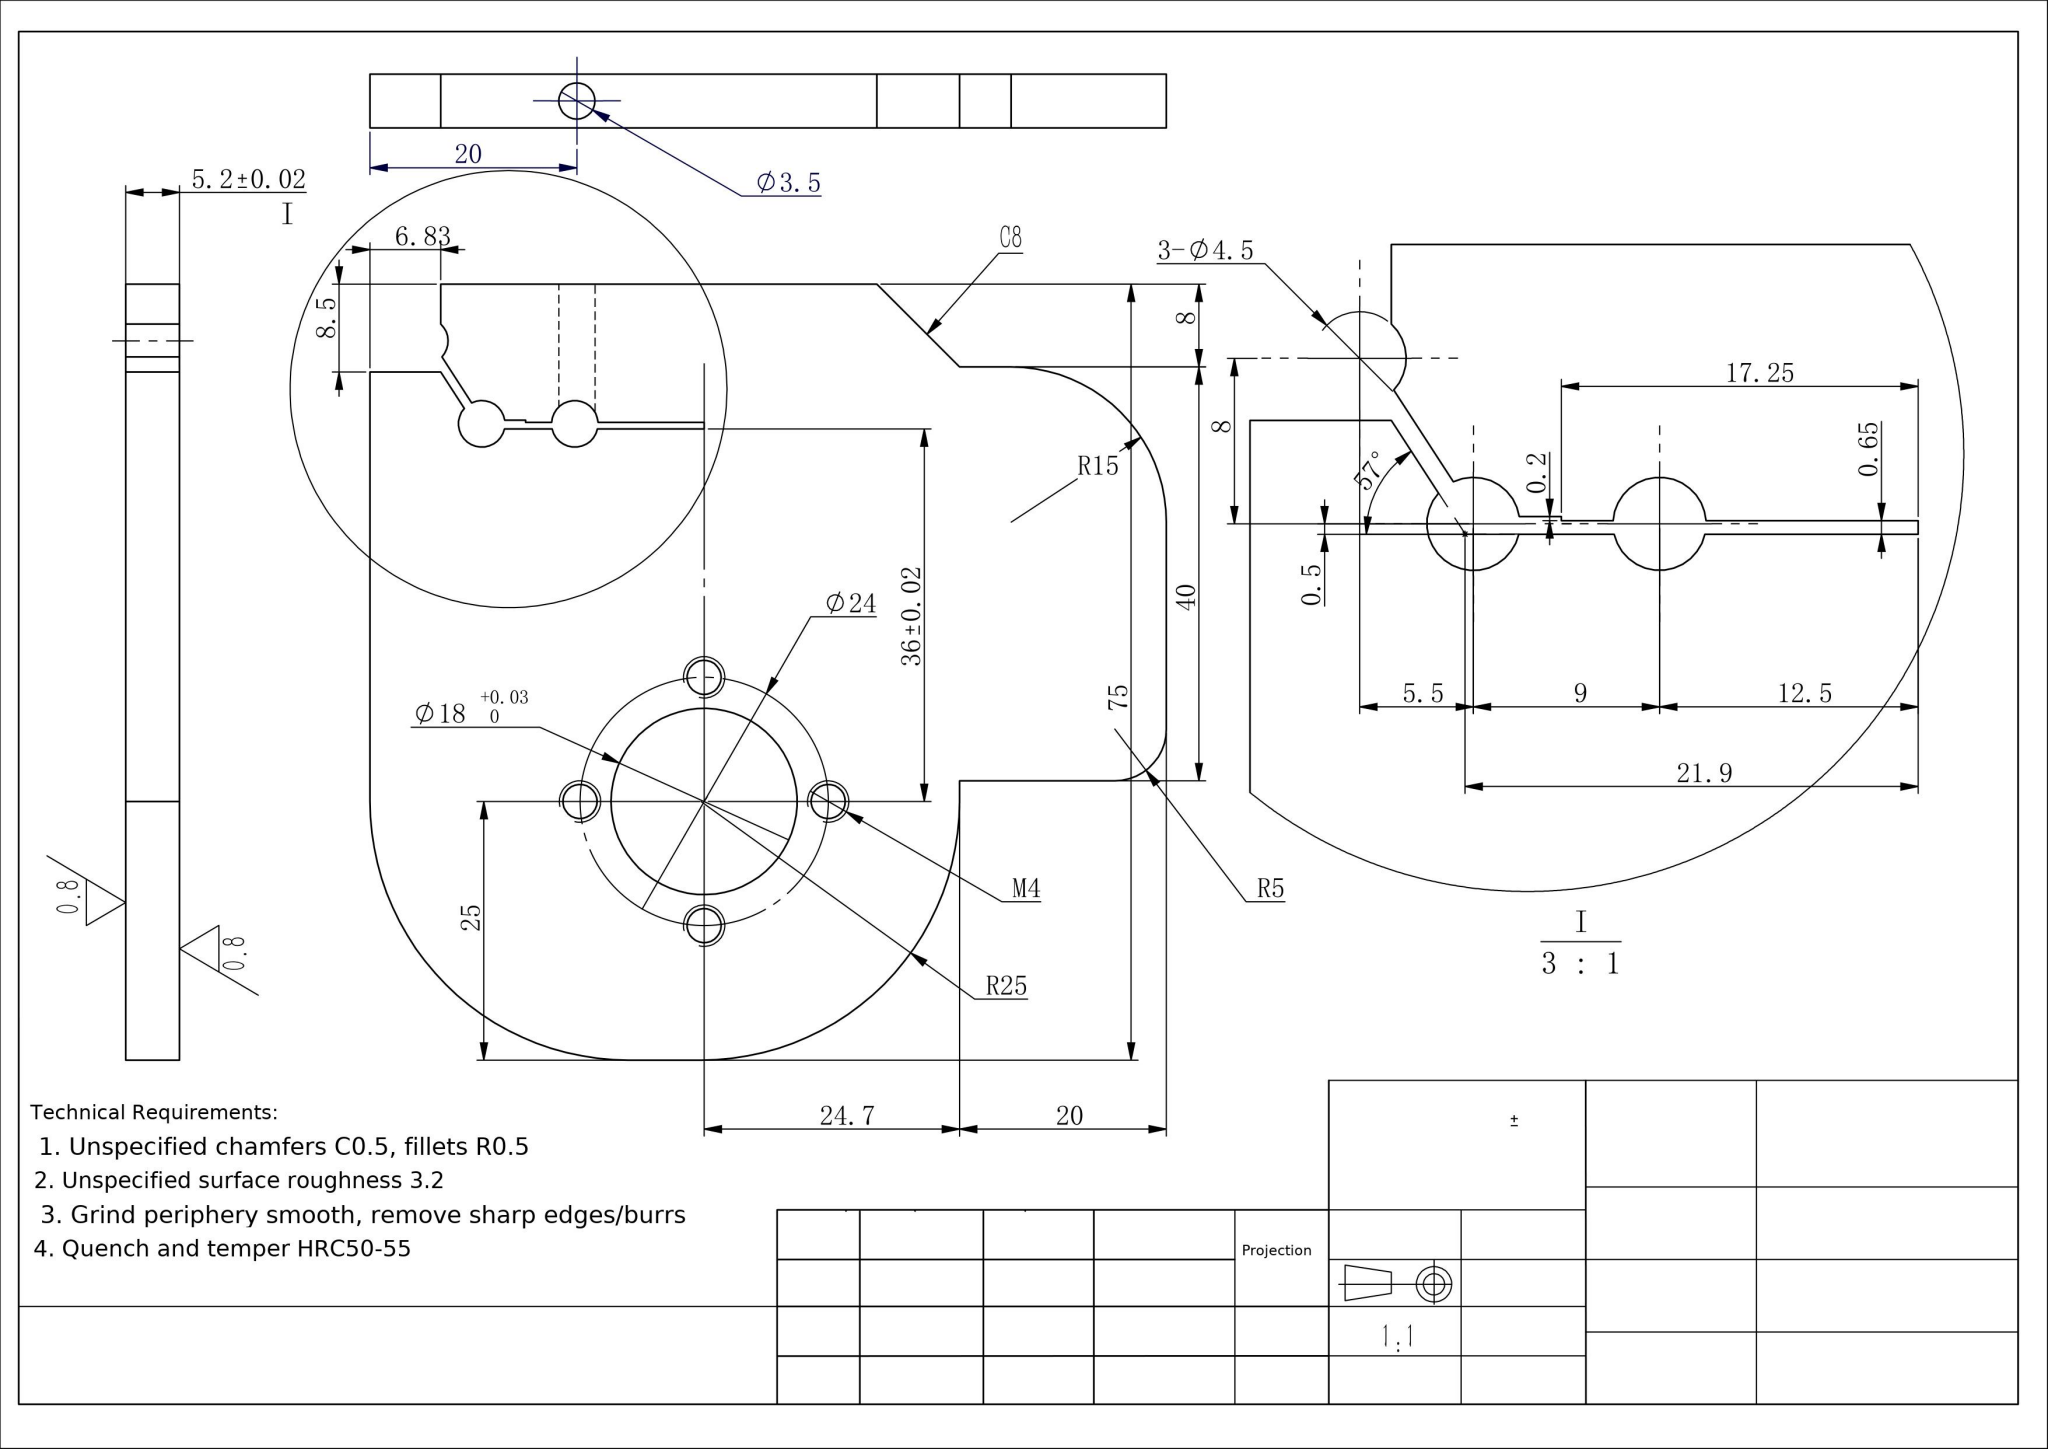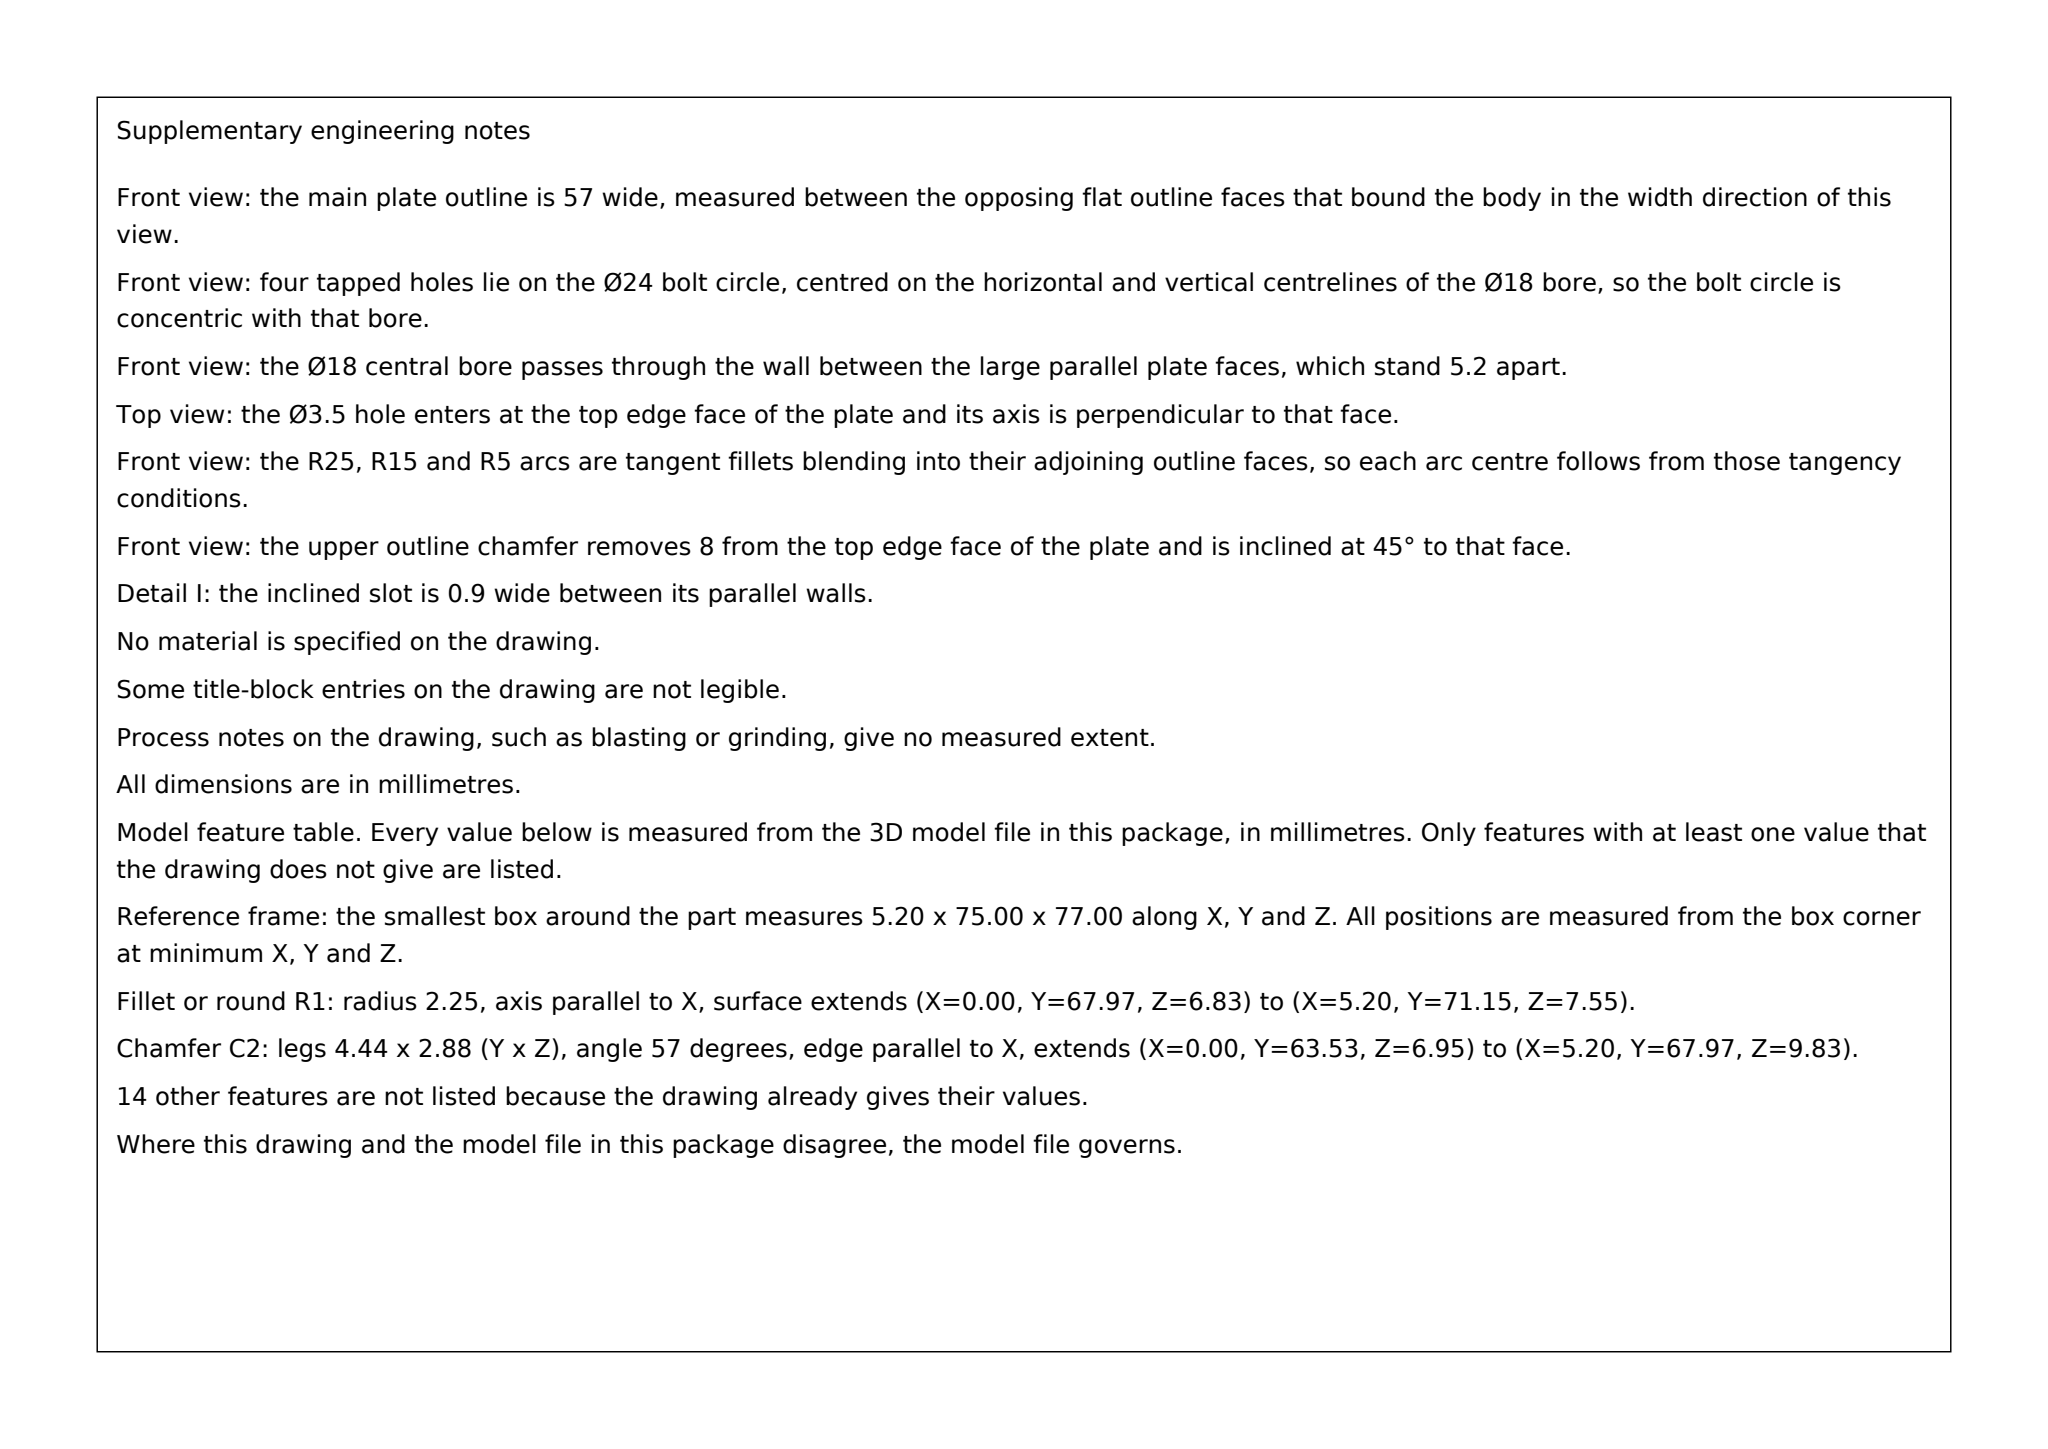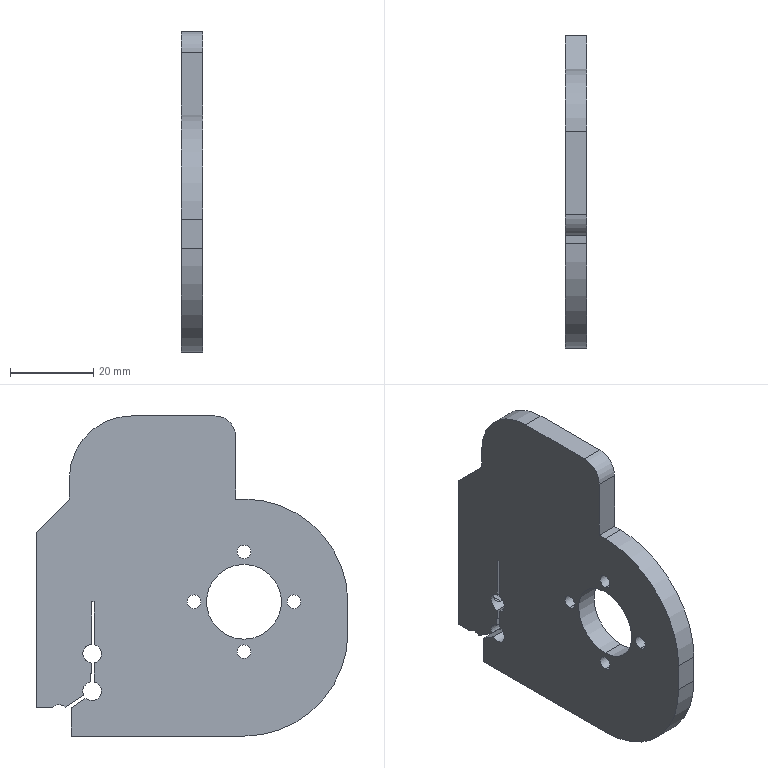Part | SolidWorks | mm | 1 solid | 43 faces | box 5.2 x 75 x 77 mm | volume 22388 mm3 | cylinder 22 | plane 21 | commonest cylinder face diameters 3.3 x8 4.5 x6 3.5 x2 18 x2 50 x2 10 x1 30 x1
Drawing notes:
4X M4 TAPPED HOLE THRU (Ø3.3 tap drill, 5.2 plate thickness) | from the solid: four Ø3.3 cylinders, axis x, length 5.2 = bbox x (5.2) = through plate
M4 holes equally spaced 90° apart on the Ø24 B.C.; axes at Y13.0/Z32.3, Y37.0/Z32.3, Y25.0/Z20.3, Y25.0/Z44.3 from the bbox min corner | from the solid: cylinders[3.3,x] positions [13,32.3],[37,32.3],[25,20.3],[25,44.3]
Ø18 +0.03/0 bore THRU; axis located 32.3 from the Z=0 outline edge and 25 from the Y=0 bottom edge | from the solid: cylinder [18.0,'x',[null,25.0,32.3],5.2]; planes z=0 and y=0
The 36±0.02 is taken from the Y=61 horizontal face to the Ø18 bore axis (25 + 36 = 61) | from the solid: axis_plane y=61.0 and Ø18 axis at y=25.0
Ø3.5 hole drilled from the Y=75 end face, depth 12.38 (blind); axis 20 from the Z=0 edge and 2.6 from the X=0 face (mid-thickness) | from the solid: cylinder [3.5,'y',[2.6,null,20.0],12.38]; plane y=75.0
3X Ø4.5 THRU, axes normal to the 5.2 plate faces, at Y61.5/Z10.8, Y61.5/Z19.8 and Y69.5/Z5.3 from the bbox min corner | from the solid: cylinders [4.5,'x',[null,61.5,10.8]], [4.5,'x',[null,61.5,19.8]], [4.5,'x',[null,69.5,5.3]], each length 5.2
Detail I groove located from datums: profile steps at Z=6.83 and Z=15.05 from the Z=0 edge; groove faces at Y=61.65, 61.85, 66.5 and 67.0 from the Y=0 edge | from the solid: axis_planes z=6.83, z=15.05 and y=61.65, 61.85, 66.5, 67.0
Overall part envelope 77 (Z) x 75 (Y) x 5.2 (X) thick | from the solid: bbox_xyz [5.2,75.0,77.0]
R25 outline arc centre is at Y=25, Z=25 - NOT coincident with the Ø18 bore axis (Z=32.3) | from the solid: cylinder [50.0,'x',[null,25.0,25.0],5.2] vs Ø18 axis at [null,25.0,32.3]
All dimensions in millimetres | from the solid: STEP model facts stated in mm
C8 chamfer is 8 x 8, cut between the Y=75 top face and the Y=67 face (Y measured from the Y=0 bottom edge) | from the solid: axis_planes: y=75.0 and y=67.0 (normal-Y faces); bbox_xyz Y=75.0